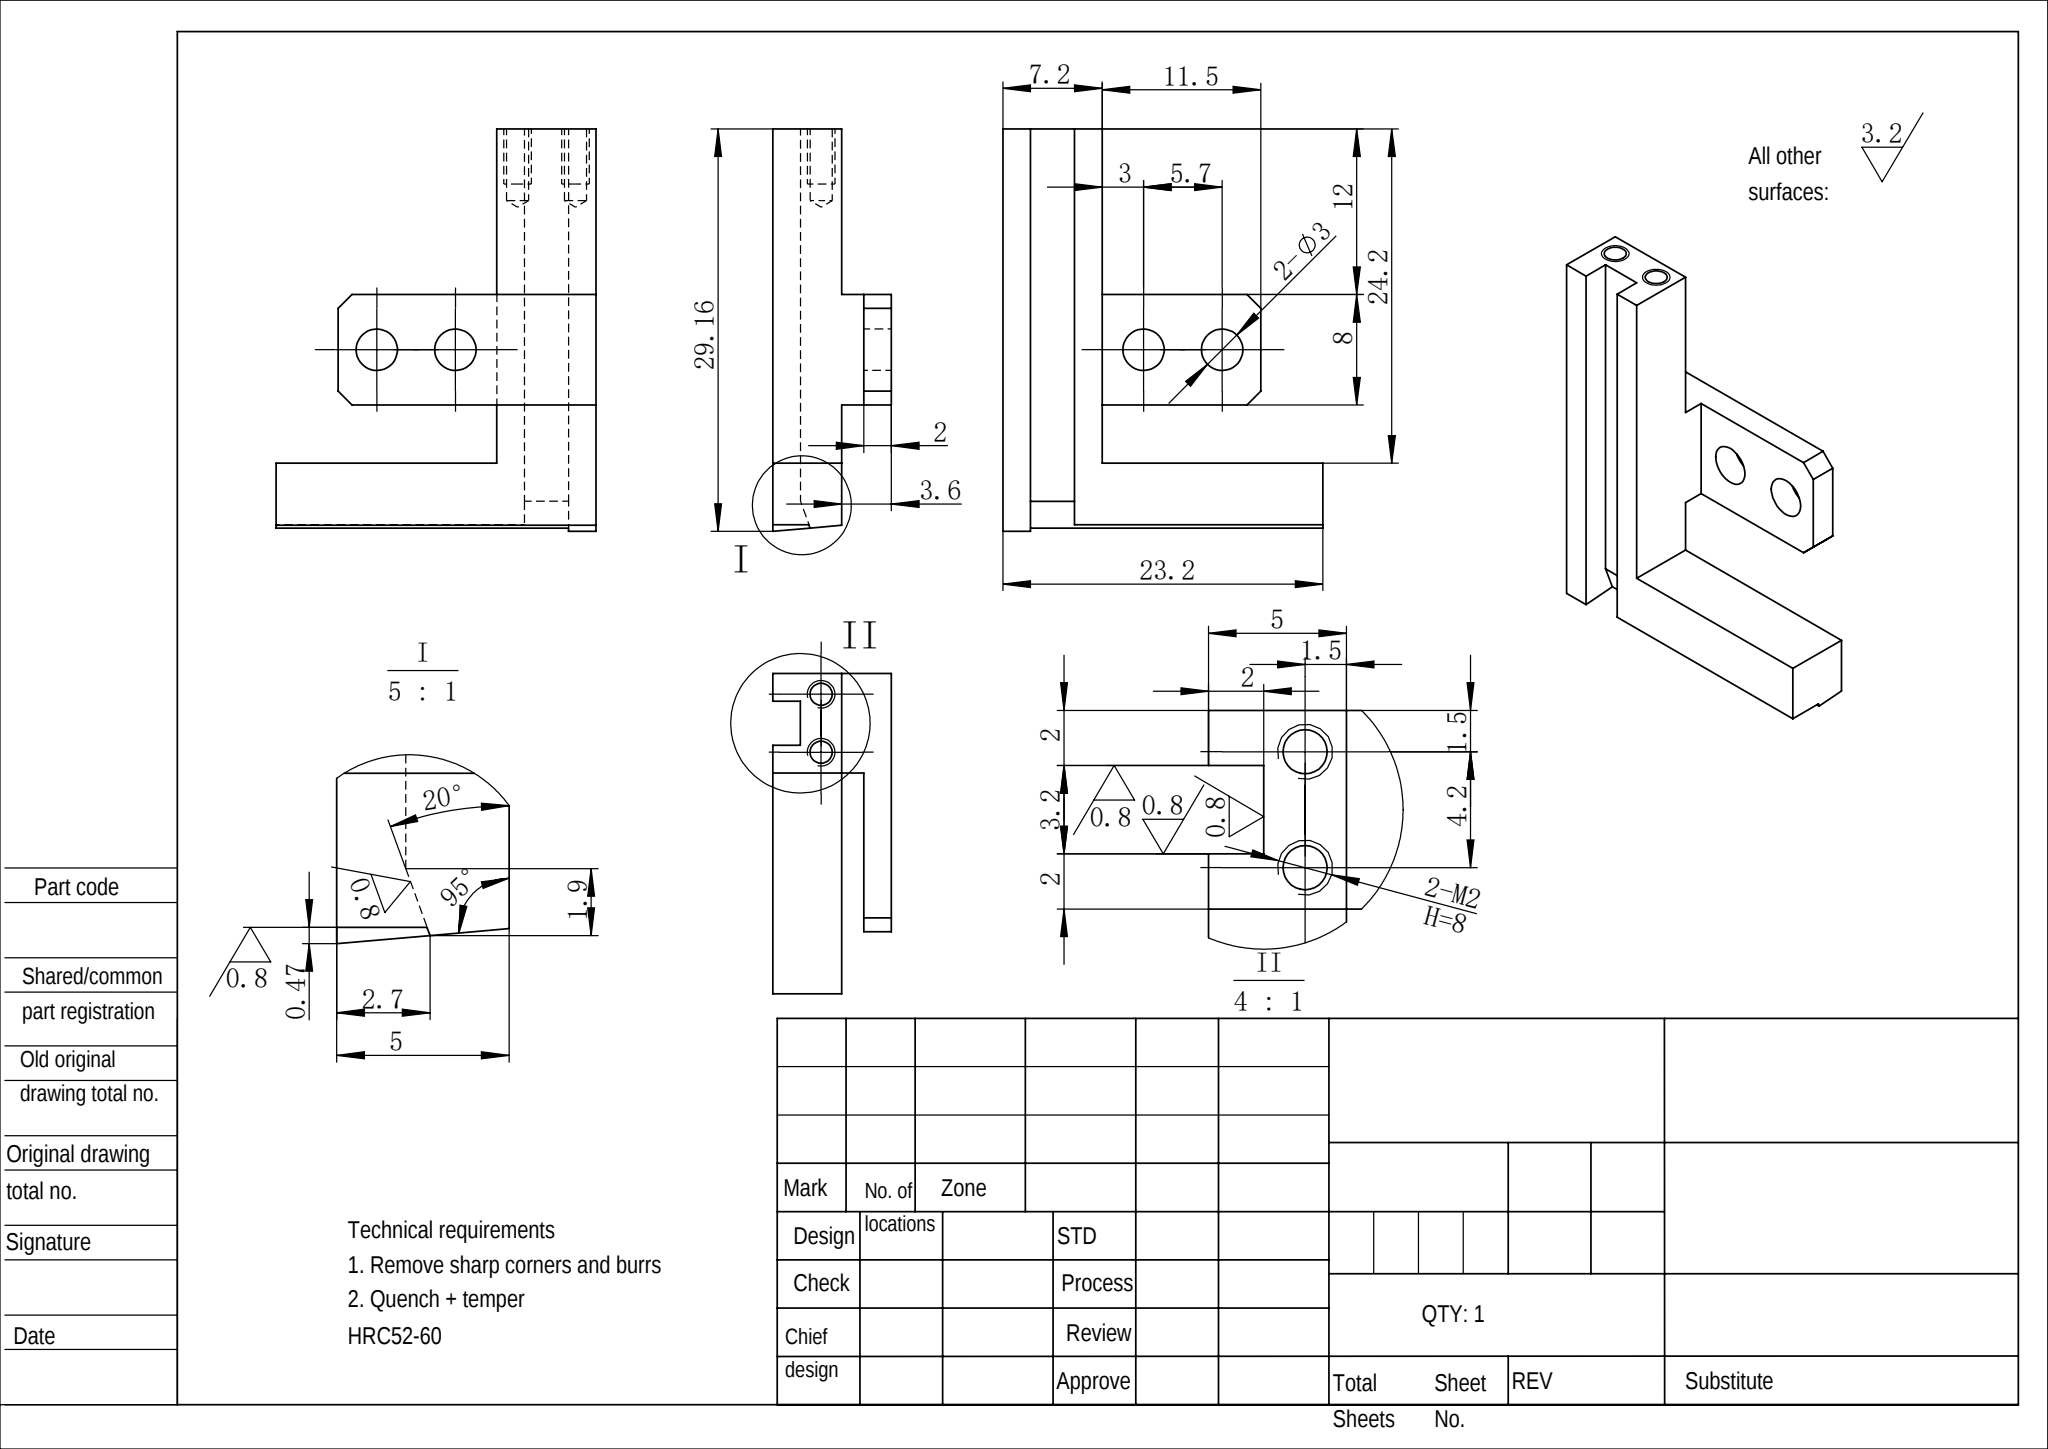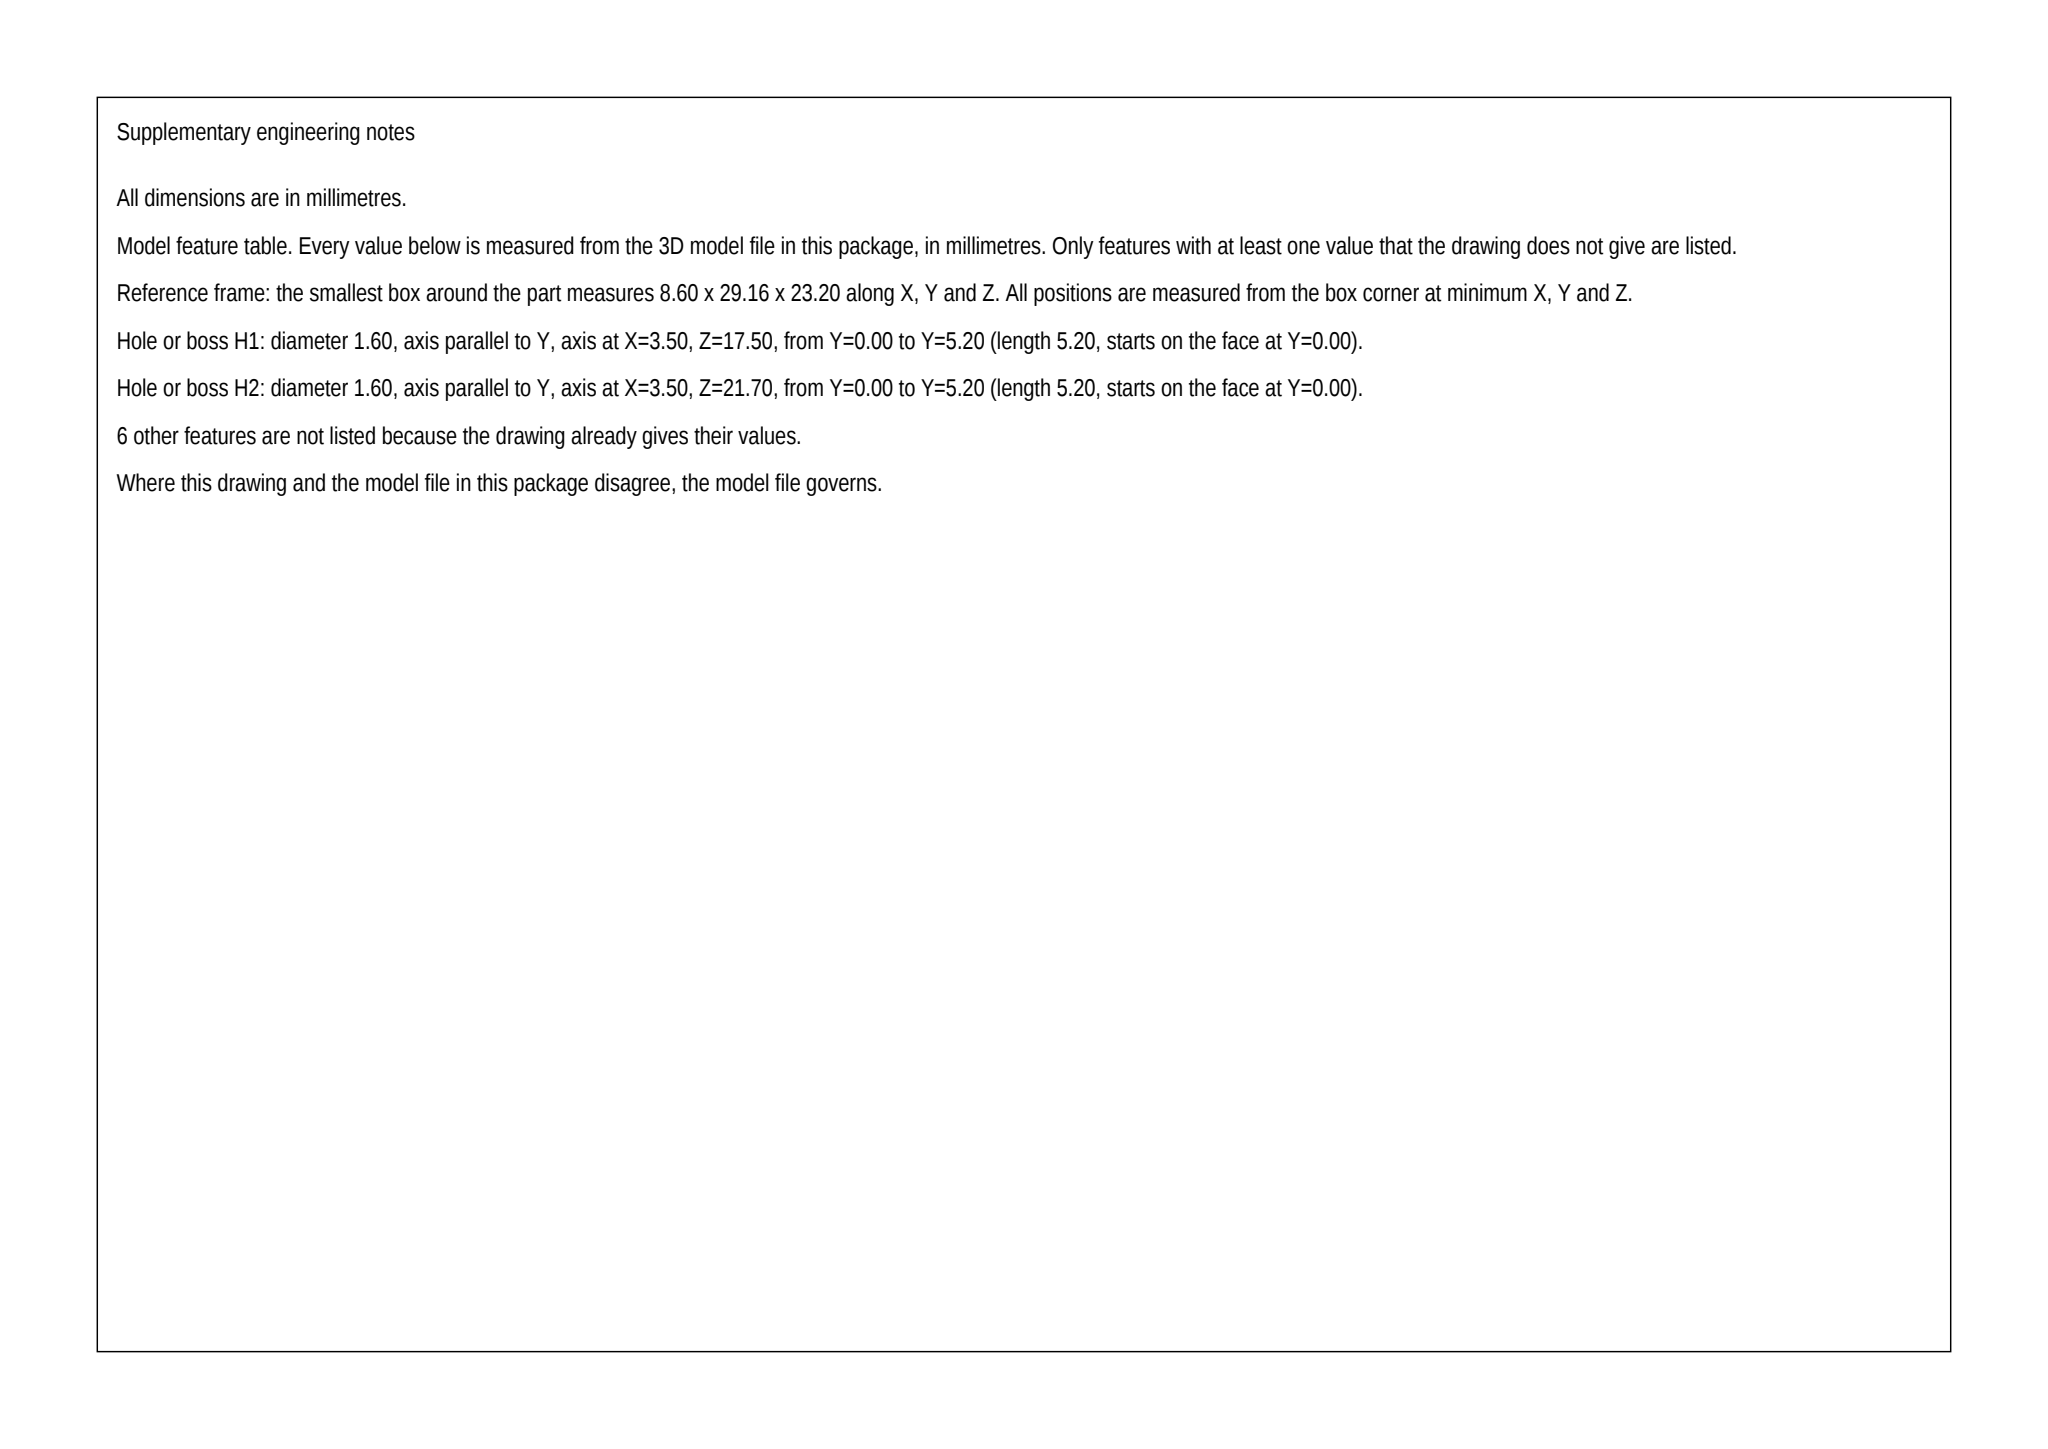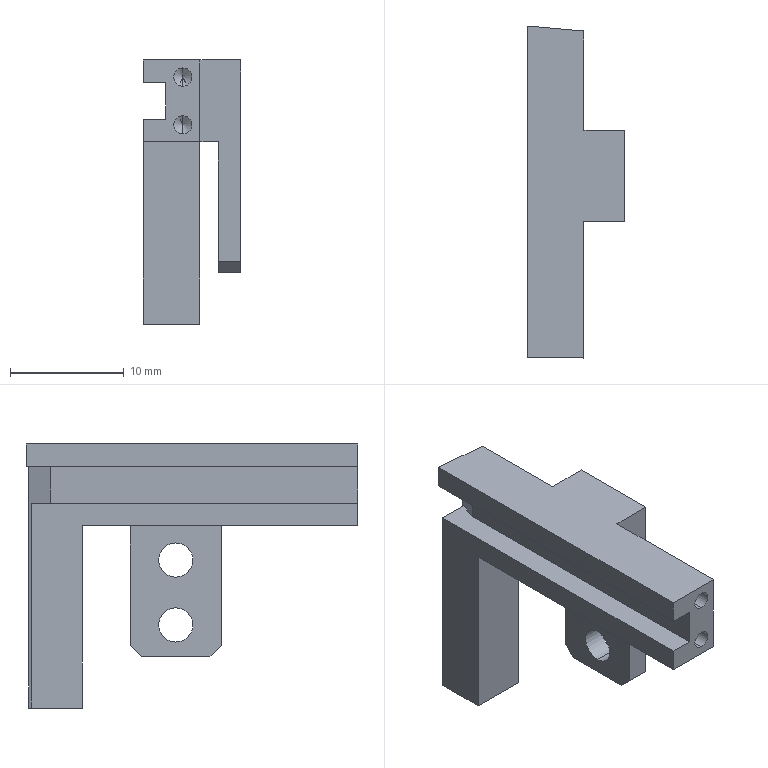Part | SolidWorks | mm | 1 solid | 34 faces | box 8.6 x 29.16 x 23.2 mm | volume 1553 mm3 | plane 22 | cylinder 8 | cone 4 | commonest cylinder face diameters 1.6 x4 3 x4